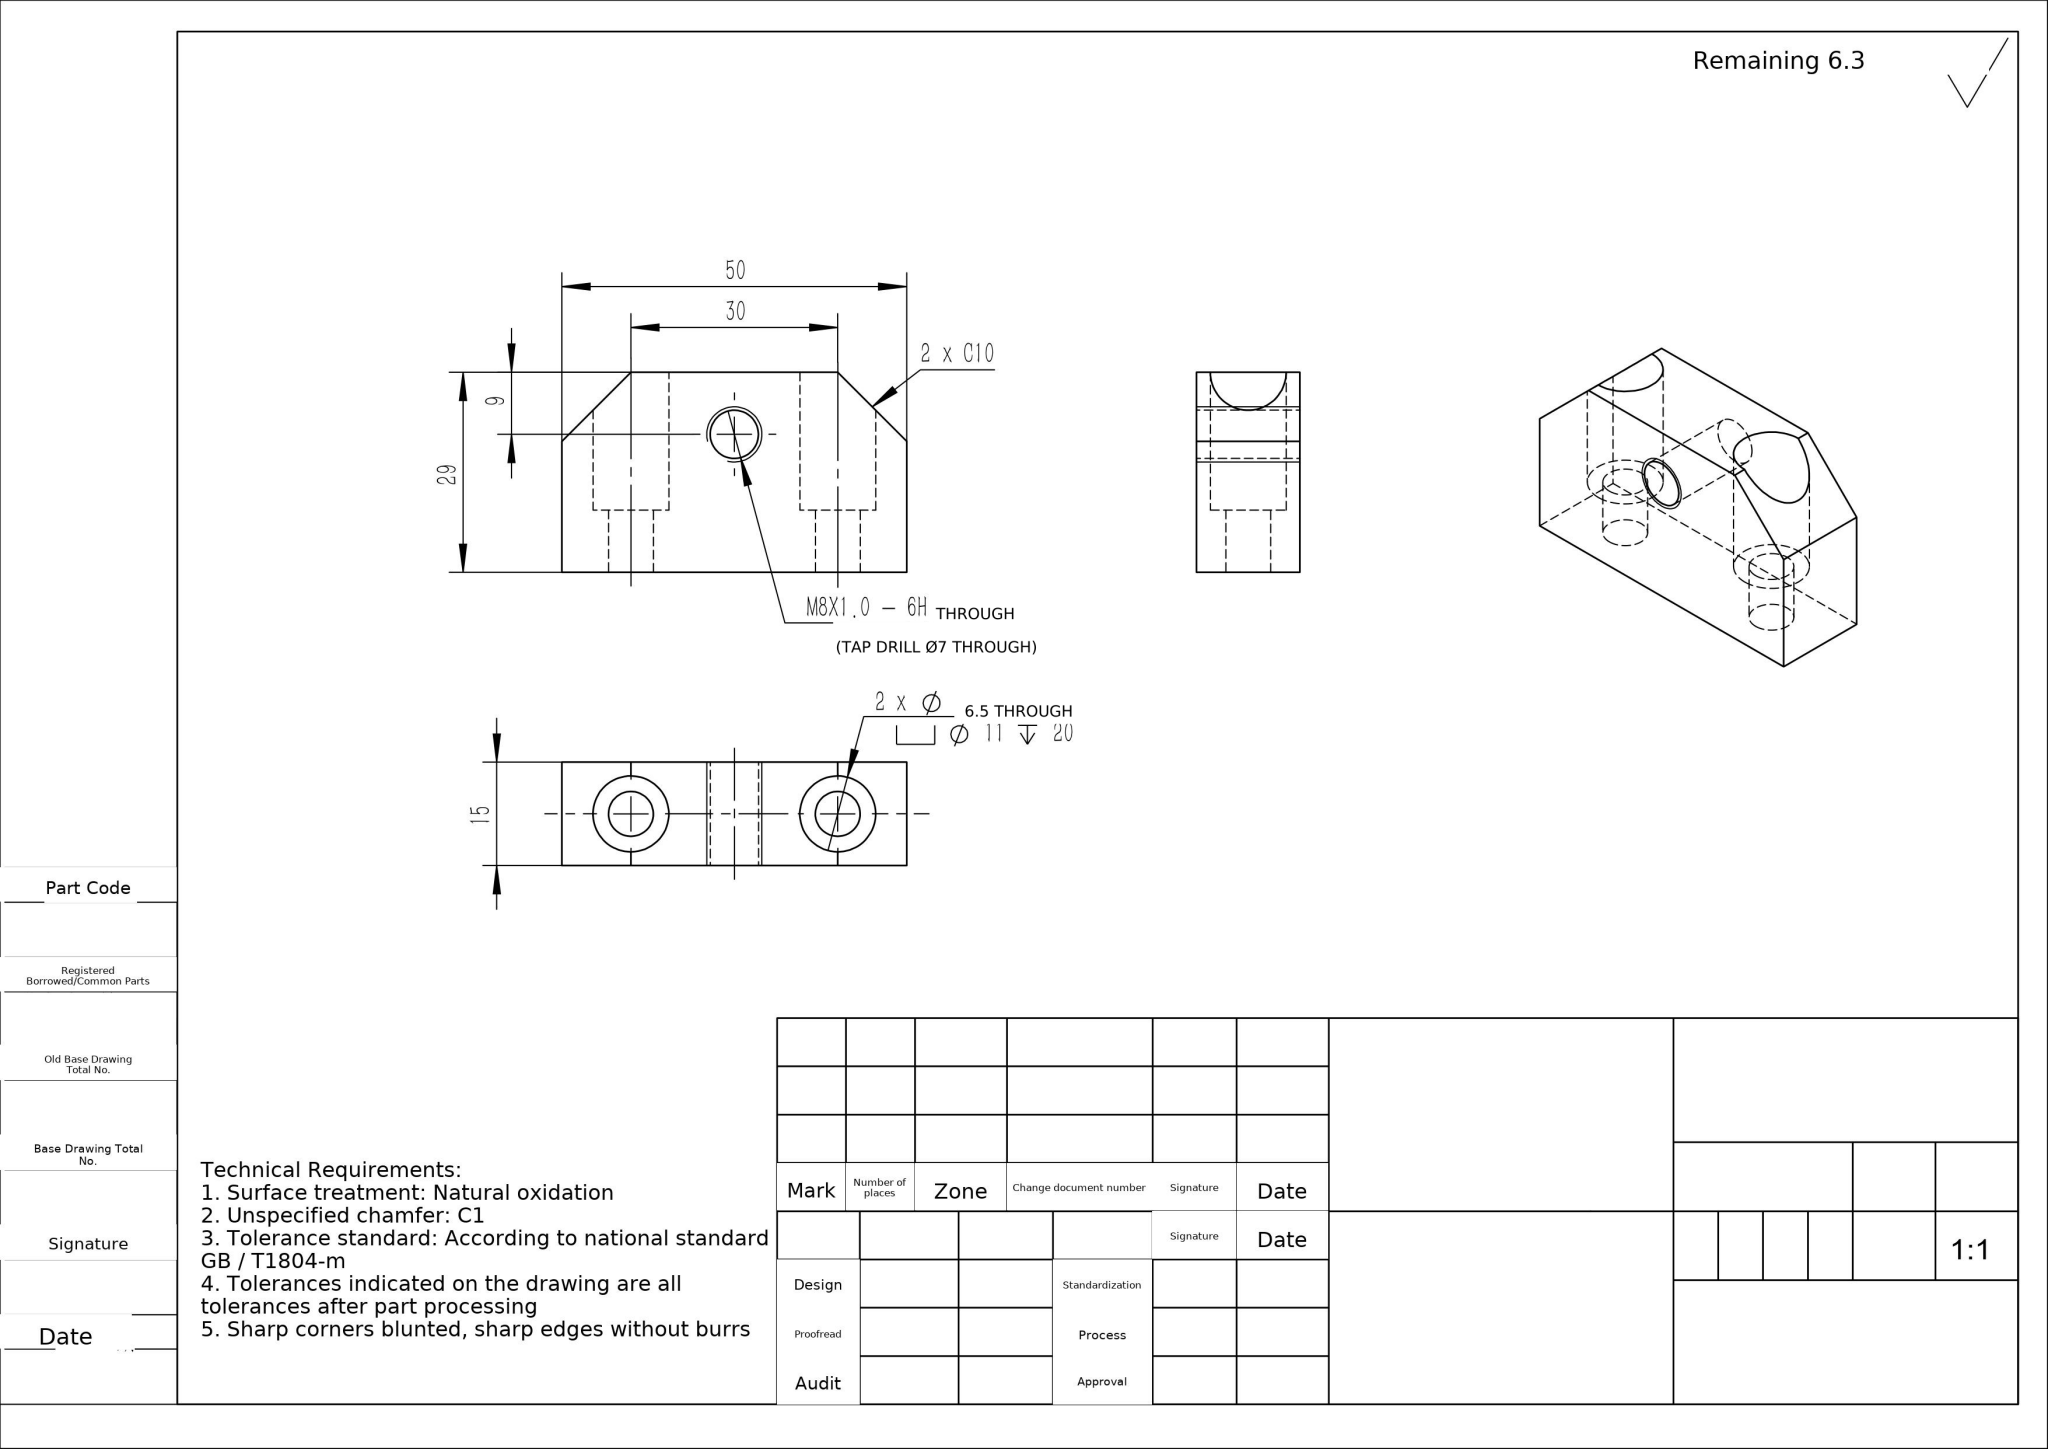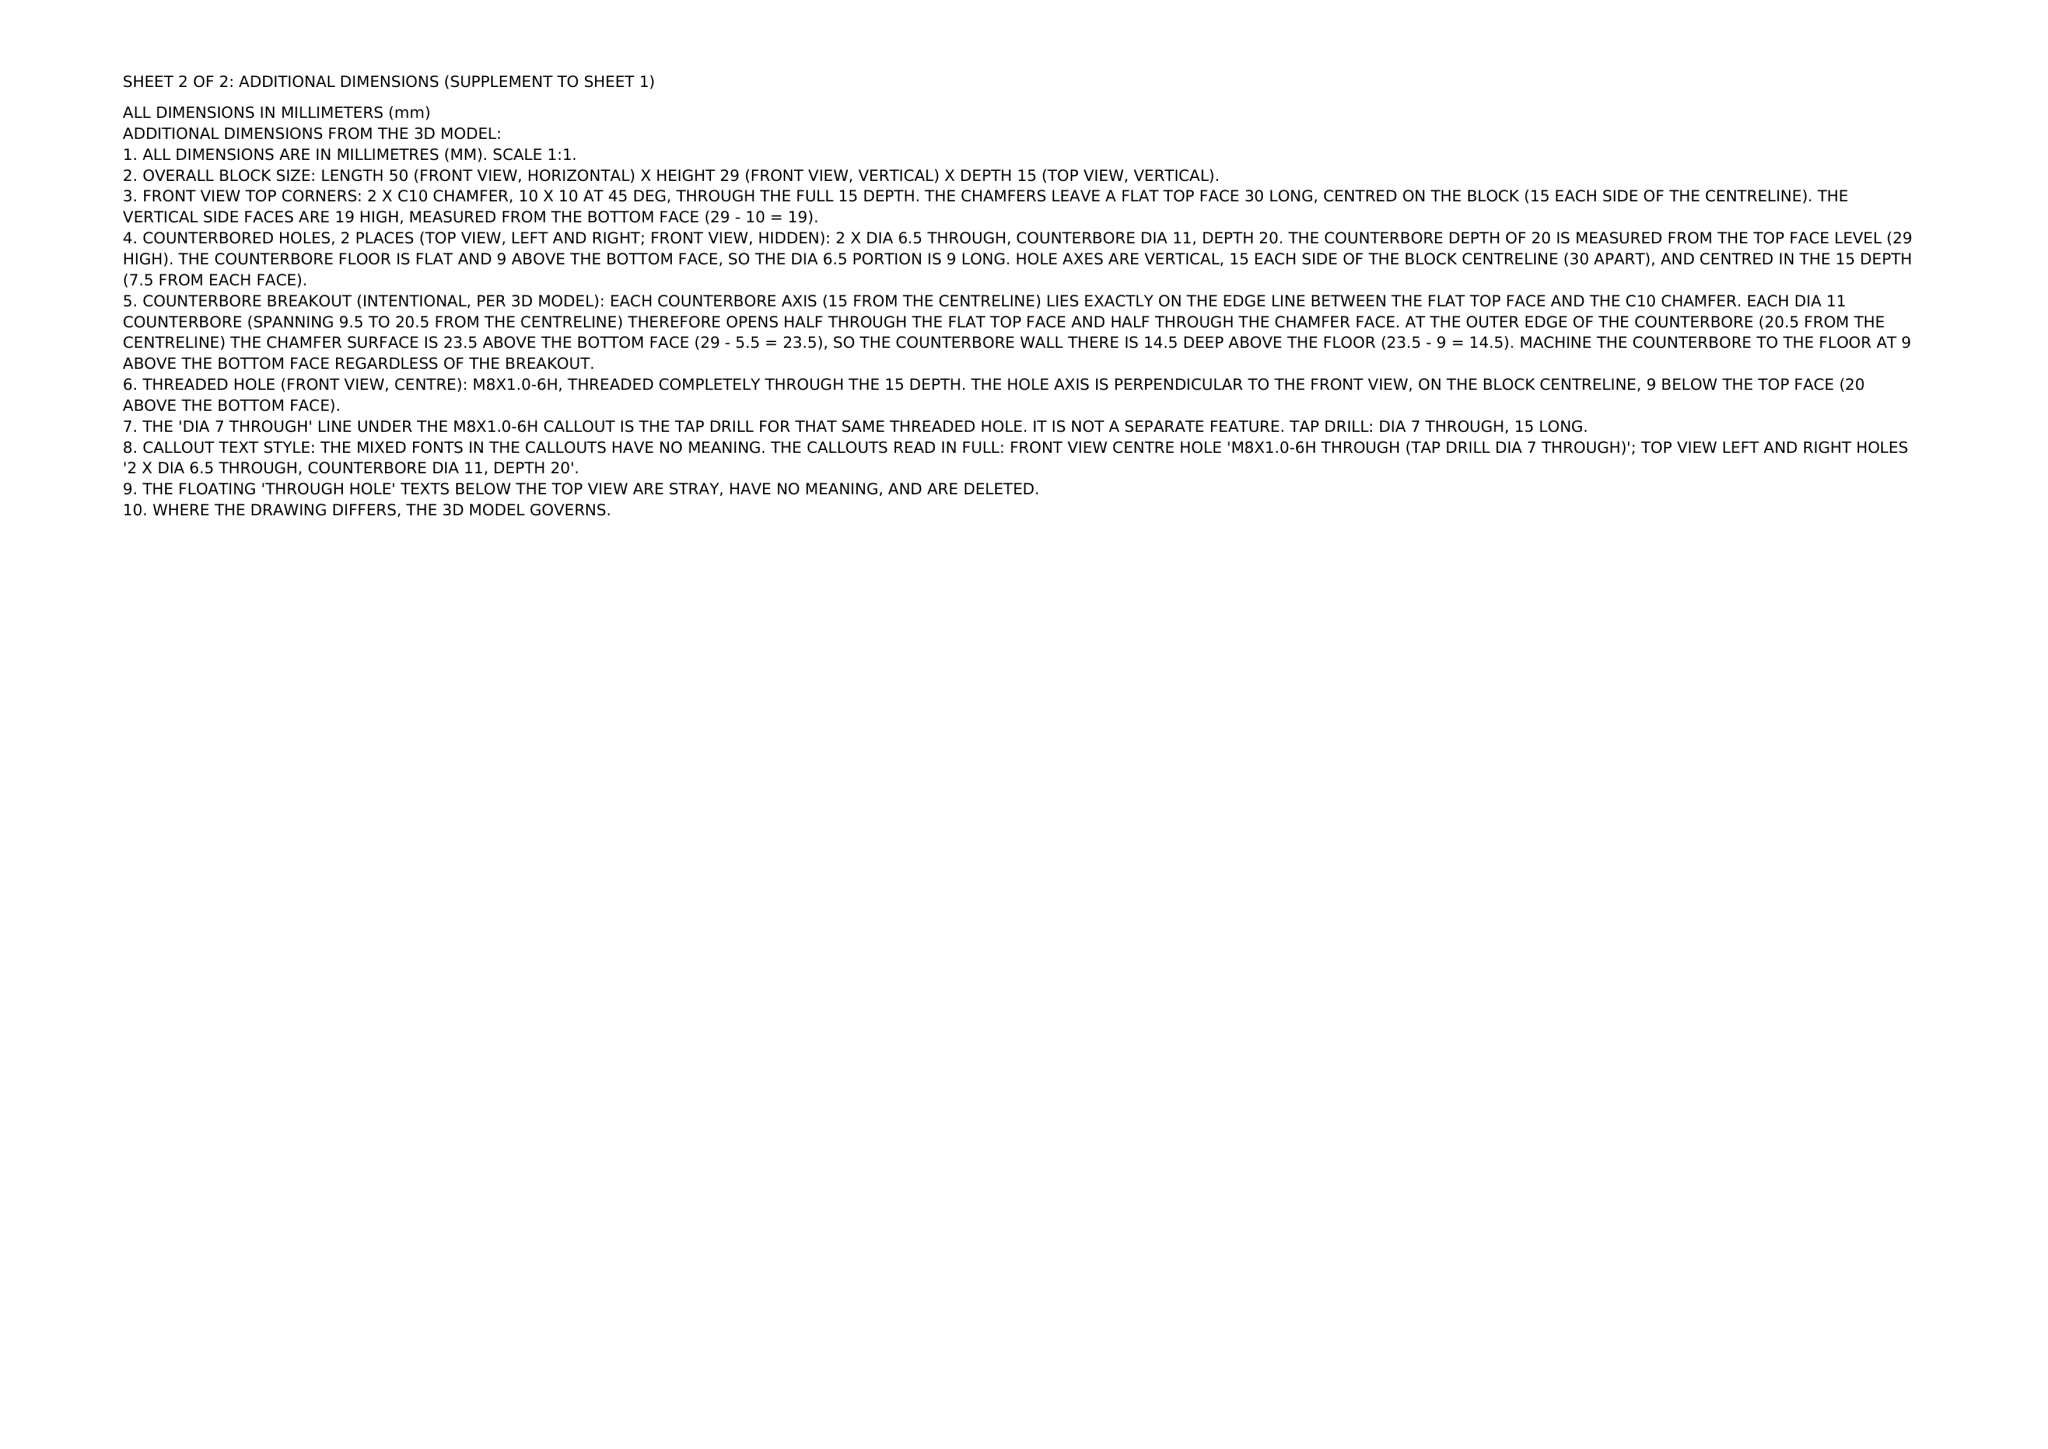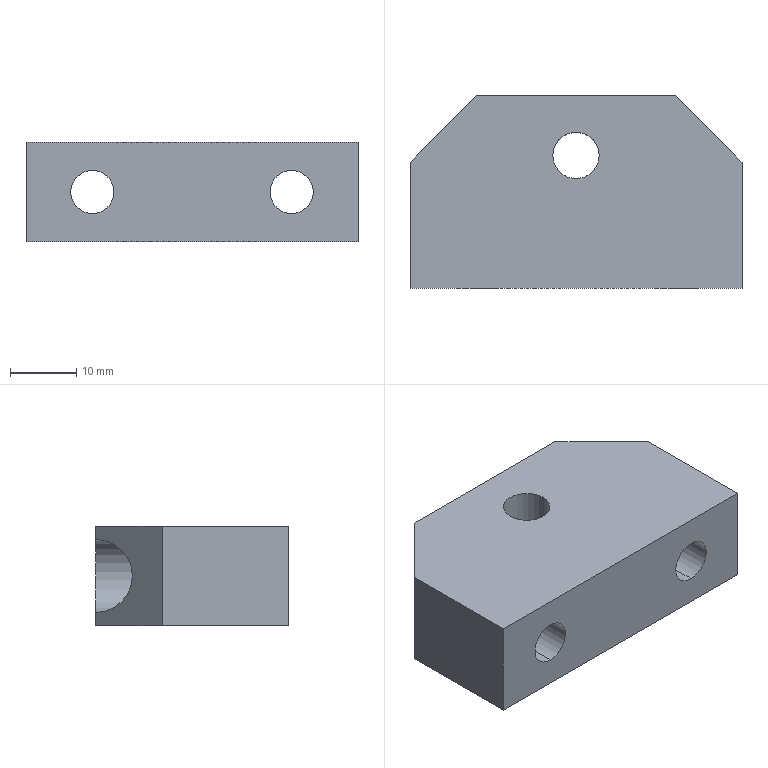Part | NX | mm | Chamfered Dual-Bore Rectangular Mounting Block | 1 solid | 20 faces | box 50 x 29 x 15 mm | volume 15496 mm3 | cylinder 10 | plane 10 | commonest cylinder face diameters 11 x4 6.5 x4 7 x2
STEP:
#1=COLOUR_RGB('',0.7922,0.8196,0.9333);
#2=FILL_AREA_STYLE_COLOUR('',#1);
#3=FILL_AREA_STYLE('',(#2));
#4=SURFACE_STYLE_FILL_AREA(#3);
#5=SURFACE_SIDE_STYLE('',(#4));
#6=SURFACE_STYLE_USAGE(.BOTH.,#5);
#7=PRESENTATION_STYLE_ASSIGNMENT((#6));
#8=CARTESIAN_POINT('',(-3.5,20.,-7.5));
#9=VERTEX_POINT('',#8);
#10=CARTESIAN_POINT('',(3.5,20.,-7.5));
#11=VERTEX_POINT('',#10);
#12=CARTESIAN_POINT('',(0.,20.,-7.5));
#13=DIRECTION('',(0.,0.,1.));
#14=DIRECTION('',(1.,0.,0.));
#15=AXIS2_PLACEMENT_3D('',#12,#13,#14);
#16=CIRCLE('',#15,3.5);
#17=EDGE_CURVE('',#9,#11,#16,.T.);
#18=ORIENTED_EDGE('',*,*,#17,.F.);
#19=CARTESIAN_POINT('',(-3.5,20.,7.5));
#20=VERTEX_POINT('',#19);
#21=CARTESIAN_POINT('',(-3.5,20.,7.5));
#22=DIRECTION('',(0.,0.,1.));
#23=VECTOR('',#22,1000.);
#24=LINE('',#21,#23);
#25=EDGE_CURVE('',#9,#20,#24,.T.);
#26=ORIENTED_EDGE('',*,*,#25,.T.);
#27=CARTESIAN_POINT('',(3.5,20.,7.5));
#28=VERTEX_POINT('',#27);
#29=CARTESIAN_POINT('',(0.,20.,7.5));
#30=DIRECTION('',(0.,0.,1.));
#31=DIRECTION('',(1.,0.,0.));
#32=AXIS2_PLACEMENT_3D('',#29,#30,#31);
#33=CIRCLE('',#32,3.5);
#34=EDGE_CURVE('',#20,#28,#33,.T.);
#35=ORIENTED_EDGE('',*,*,#34,.T.);
#36=CARTESIAN_POINT('',(3.5,20.,7.5));
#37=DIRECTION('',(0.,0.,1.));
#38=VECTOR('',#37,1000.);
#39=LINE('',#36,#38);
#40=EDGE_CURVE('',#11,#28,#39,.T.);
#41=ORIENTED_EDGE('',*,*,#40,.F.);
#42=EDGE_LOOP('',(#18,#26,#35,#41));
#43=FACE_OUTER_BOUND('',#42,.T.);
#44=CARTESIAN_POINT('',(0.,20.,7.5));
#45=DIRECTION('',(0.,0.,1.));
#46=DIRECTION('',(1.,0.,0.));
#47=AXIS2_PLACEMENT_3D('',#44,#45,#46);
#48=CYLINDRICAL_SURFACE('',#47,3.5);
#49=ADVANCED_FACE('',(#43),#48,.F.);
#50=STYLED_ITEM('',(#7),#49);
#51=PRESENTATION_LAYER_ASSIGNMENT('','',(#50));
#52=(LENGTH_UNIT()NAMED_UNIT(*)SI_UNIT(.MILLI.,.METRE.));
#53=UNCERTAINTY_MEASURE_WITH_UNIT(LENGTH_MEASURE(0.00001),#52,'','');
#54=(NAMED_UNIT(*)PLANE_ANGLE_UNIT()SI_UNIT($,.RADIAN.));
#55=(NAMED_UNIT(*)SI_UNIT($,.STERADIAN.)SOLID_ANGLE_UNIT());
#56=(GEOMETRIC_REPRESENTATION_CONTEXT(3)GLOBAL_UNCERTAINTY_ASSIGNED_CONTEXT((#53))GLOBAL_UNIT_ASSIGNED_CONTEXT((#52,#54,#55))REPRESENTATION_CONTEXT('',''));
#57=MECHANICAL_DESIGN_GEOMETRIC_PRESENTATION_REPRESENTATION('',(#50),#56);
#58=COLOUR_RGB('',0.7922,0.8196,0.9333);
#59=FILL_AREA_STYLE_COLOUR('',#58);
#60=FILL_AREA_STYLE('',(#59));
#61=SURFACE_STYLE_FILL_AREA(#60);
#62=SURFACE_SIDE_STYLE('',(#61));
#63=SURFACE_STYLE_USAGE(.BOTH.,#62);
#64=PRESENTATION_STYLE_ASSIGNMENT((#63));
#65=ORIENTED_EDGE('',*,*,#25,.F.);
#66=CARTESIAN_POINT('',(0.,20.,-7.5));
#67=DIRECTION('',(0.,0.,1.));
#68=DIRECTION('',(1.,0.,0.));
#69=AXIS2_PLACEMENT_3D('',#66,#67,#68);
#70=CIRCLE('',#69,3.5);
#71=EDGE_CURVE('',#11,#9,#70,.T.);
#72=ORIENTED_EDGE('',*,*,#71,.F.);
#73=ORIENTED_EDGE('',*,*,#40,.T.);
#74=CARTESIAN_POINT('',(0.,20.,7.5));
#75=DIRECTION('',(0.,0.,1.));
#76=DIRECTION('',(1.,0.,0.));
#77=AXIS2_PLACEMENT_3D('',#74,#75,#76);
#78=CIRCLE('',#77,3.5);
#79=EDGE_CURVE('',#28,#20,#78,.T.);
#80=ORIENTED_EDGE('',*,*,#79,.T.);
#81=EDGE_LOOP('',(#65,#72,#73,#80));
#82=FACE_OUTER_BOUND('',#81,.T.);
#83=CARTESIAN_POINT('',(0.,20.,7.5));
#84=DIRECTION('',(0.,0.,1.));
#85=DIRECTION('',(1.,0.,0.));
#86=AXIS2_PLACEMENT_3D('',#83,#84,#85);
#87=CYLINDRICAL_SURFACE('',#86,3.5);
#88=ADVANCED_FACE('',(#82),#87,.F.);
#89=STYLED_ITEM('',(#64),#88);
#90=PRESENTATION_LAYER_ASSIGNMENT('','',(#89));
#91=COLOUR_RGB('',1.,0.3725,0.6118);
#92=FILL_AREA_STYLE_COLOUR('',#91);
#93=FILL_AREA_STYLE('',(#92));
#94=SURFACE_STYLE_FILL_AREA(#93);
#95=SURFACE_SIDE_STYLE('',(#94));
#96=SURFACE_STYLE_USAGE(.BOTH.,#95);
#97=PRESENTATION_STYLE_ASSIGNMENT((#96));
#98=CARTESIAN_POINT('',(-15.,9.,-5.5));
#99=VERTEX_POINT('',#98);
#100=CARTESIAN_POINT('',(-15.,9.,5.5));
#101=VERTEX_POINT('',#100);
#102=CARTESIAN_POINT('',(-15.,9.,0.));
#103=DIRECTION('',(0.,1.,0.));
#104=DIRECTION('',(0.,0.,1.));
#105=AXIS2_PLACEMENT_3D('',#102,#103,#104);
#106=CIRCLE('',#105,5.5);
#107=EDGE_CURVE('',#99,#101,#106,.T.);
#108=ORIENTED_EDGE('',*,*,#107,.F.);
#109=CARTESIAN_POINT('',(-15.,29.,-5.5));
#110=VERTEX_POINT('',#109);
#111=CARTESIAN_POINT('',(-15.,29.,-5.5));
#112=DIRECTION('',(0.,1.,0.));
#113=VECTOR('',#112,1000.);
#114=LINE('',#111,#113);
#115=EDGE_CURVE('',#99,#110,#114,.T.);
#116=ORIENTED_EDGE('',*,*,#115,.T.);
#117=CARTESIAN_POINT('',(-15.,29.,5.5));
#118=VERTEX_POINT('',#117);
#119=CARTESIAN_POINT('',(-15.,29.,-5.5));
#120=CARTESIAN_POINT('',(-26.,18.,-5.5));
#121=CARTESIAN_POINT('',(-26.,18.,5.5));
#122=CARTESIAN_POINT('',(-15.,29.,5.5));
#123=(BOUNDED_CURVE()B_SPLINE_CURVE(3,(#119,#120,#121,#122),.UNSPECIFIED.,.F.,.T.)B_SPLINE_CURVE_WITH_KNOTS((4,4),(1.571,4.712),.UNSPECIFIED.)CURVE()GEOMETRIC_REPRESENTATION_ITEM()RATIONAL_B_SPLINE_CURVE((1.,0.3333,0.3333,1.))REPRESENTATION_ITEM(''));
#124=EDGE_CURVE('',#110,#118,#123,.T.);
#125=ORIENTED_EDGE('',*,*,#124,.T.);
#126=CARTESIAN_POINT('',(-15.,29.,5.5));
#127=DIRECTION('',(0.,1.,0.));
#128=VECTOR('',#127,1000.);
#129=LINE('',#126,#128);
#130=EDGE_CURVE('',#101,#118,#129,.T.);
#131=ORIENTED_EDGE('',*,*,#130,.F.);
#132=EDGE_LOOP('',(#108,#116,#125,#131));
#133=FACE_OUTER_BOUND('',#132,.T.);
#134=CARTESIAN_POINT('',(-15.,29.,0.));
#135=DIRECTION('',(0.,1.,0.));
#136=DIRECTION('',(0.,0.,1.));
#137=AXIS2_PLACEMENT_3D('',#134,#135,#136);
#138=CYLINDRICAL_SURFACE('',#137,5.5);
#139=ADVANCED_FACE('',(#133),#138,.F.);
#140=CARTESIAN_POINT('',(-15.,0.,-3.25));
#141=VERTEX_POINT('',#140);
#142=CARTESIAN_POINT('',(-15.,0.,3.25));
#143=VERTEX_POINT('',#142);
#144=CARTESIAN_POINT('',(-15.,0.,0.));
#145=DIRECTION('',(0.,1.,0.));
#146=DIRECTION('',(0.,0.,1.));
#147=AXIS2_PLACEMENT_3D('',#144,#145,#146);
#148=CIRCLE('',#147,3.25);
#149=EDGE_CURVE('',#141,#143,#148,.T.);
#150=ORIENTED_EDGE('',*,*,#149,.F.);
#151=CARTESIAN_POINT('',(-15.,9.,-3.25));
#152=VERTEX_POINT('',#151);
#153=CARTESIAN_POINT('',(-15.,29.,-3.25));
#154=DIRECTION('',(0.,1.,0.));
#155=VECTOR('',#154,1000.);
#156=LINE('',#153,#155);
#157=EDGE_CURVE('',#141,#152,#156,.T.);
#158=ORIENTED_EDGE('',*,*,#157,.T.);
#159=CARTESIAN_POINT('',(-15.,9.,3.25));
#160=VERTEX_POINT('',#159);
#161=CARTESIAN_POINT('',(-15.,9.,0.));
#162=DIRECTION('',(0.,1.,0.));
#163=DIRECTION('',(0.,0.,1.));
#164=AXIS2_PLACEMENT_3D('',#161,#162,#163);
#165=CIRCLE('',#164,3.25);
#166=EDGE_CURVE('',#152,#160,#165,.T.);
#167=ORIENTED_EDGE('',*,*,#166,.T.);
#168=CARTESIAN_POINT('',(-15.,29.,3.25));
#169=DIRECTION('',(0.,1.,0.));
#170=VECTOR('',#169,1000.);
#171=LINE('',#168,#170);
#172=EDGE_CURVE('',#143,#160,#171,.T.);
#173=ORIENTED_EDGE('',*,*,#172,.F.);
#174=EDGE_LOOP('',(#150,#158,#167,#173));
#175=FACE_OUTER_BOUND('',#174,.T.);
#176=CARTESIAN_POINT('',(-15.,29.,0.));
#177=DIRECTION('',(0.,1.,0.));
#178=DIRECTION('',(0.,0.,1.));
#179=AXIS2_PLACEMENT_3D('',#176,#177,#178);
#180=CYLINDRICAL_SURFACE('',#179,3.25);
#181=ADVANCED_FACE('',(#175),#180,.F.);
#182=CARTESIAN_POINT('',(15.,9.,-5.5));
#183=VERTEX_POINT('',#182);
#184=CARTESIAN_POINT('',(15.,9.,5.5));
#185=VERTEX_POINT('',#184);
#186=CARTESIAN_POINT('',(15.,9.,0.));
#187=DIRECTION('',(0.,1.,0.));
#188=DIRECTION('',(0.,0.,1.));
#189=AXIS2_PLACEMENT_3D('',#186,#187,#188);
#190=CIRCLE('',#189,5.5);
#191=EDGE_CURVE('',#183,#185,#190,.T.);
#192=ORIENTED_EDGE('',*,*,#191,.F.);
#193=CARTESIAN_POINT('',(15.,29.,-5.5));
#194=VERTEX_POINT('',#193);
#195=CARTESIAN_POINT('',(15.,29.,-5.5));
#196=DIRECTION('',(0.,1.,0.));
#197=VECTOR('',#196,1000.);
#198=LINE('',#195,#197);
#199=EDGE_CURVE('',#183,#194,#198,.T.);
#200=ORIENTED_EDGE('',*,*,#199,.T.);
#201=CARTESIAN_POINT('',(15.,29.,5.5));
#202=VERTEX_POINT('',#201);
#203=CARTESIAN_POINT('',(15.,29.,0.));
#204=DIRECTION('',(0.,1.,0.));
#205=DIRECTION('',(0.,0.,1.));
#206=AXIS2_PLACEMENT_3D('',#203,#204,#205);
#207=CIRCLE('',#206,5.5);
#208=EDGE_CURVE('',#194,#202,#207,.T.);
#209=ORIENTED_EDGE('',*,*,#208,.T.);
#210=CARTESIAN_POINT('',(15.,29.,5.5));
#211=DIRECTION('',(0.,1.,0.));
#212=VECTOR('',#211,1000.);
#213=LINE('',#210,#212);
#214=EDGE_CURVE('',#185,#202,#213,.T.);
#215=ORIENTED_EDGE('',*,*,#214,.F.);
#216=EDGE_LOOP('',(#192,#200,#209,#215));
#217=FACE_OUTER_BOUND('',#216,.T.);
#218=CARTESIAN_POINT('',(15.,29.,0.));
#219=DIRECTION('',(0.,1.,0.));
#220=DIRECTION('',(0.,0.,1.));
#221=AXIS2_PLACEMENT_3D('',#218,#219,#220);
#222=CYLINDRICAL_SURFACE('',#221,5.5);
#223=ADVANCED_FACE('',(#217),#222,.F.);
#224=CARTESIAN_POINT('',(15.,0.,-3.25));
#225=VERTEX_POINT('',#224);
#226=CARTESIAN_POINT('',(15.,0.,3.25));
#227=VERTEX_POINT('',#226);
#228=CARTESIAN_POINT('',(15.,0.,0.));
#229=DIRECTION('',(0.,1.,0.));
#230=DIRECTION('',(0.,0.,1.));
#231=AXIS2_PLACEMENT_3D('',#228,#229,#230);
#232=CIRCLE('',#231,3.25);
#233=EDGE_CURVE('',#225,#227,#232,.T.);
#234=ORIENTED_EDGE('',*,*,#233,.F.);
#235=CARTESIAN_POINT('',(15.,9.,-3.25));
#236=VERTEX_POINT('',#235);
#237=CARTESIAN_POINT('',(15.,29.,-3.25));
#238=DIRECTION('',(0.,1.,0.));
#239=VECTOR('',#238,1000.);
#240=LINE('',#237,#239);
#241=EDGE_CURVE('',#225,#236,#240,.T.);
#242=ORIENTED_EDGE('',*,*,#241,.T.);
#243=CARTESIAN_POINT('',(15.,9.,3.25));
#244=VERTEX_POINT('',#243);
#245=CARTESIAN_POINT('',(15.,9.,0.));
#246=DIRECTION('',(0.,1.,0.));
#247=DIRECTION('',(0.,0.,1.));
#248=AXIS2_PLACEMENT_3D('',#245,#246,#247);
#249=CIRCLE('',#248,3.25);
#250=EDGE_CURVE('',#236,#244,#249,.T.);
#251=ORIENTED_EDGE('',*,*,#250,.T.);
#252=CARTESIAN_POINT('',(15.,29.,3.25));
#253=DIRECTION('',(0.,1.,0.));
#254=VECTOR('',#253,1000.);
#255=LINE('',#252,#254);
#256=EDGE_CURVE('',#227,#244,#255,.T.);
#257=ORIENTED_EDGE('',*,*,#256,.F.);
#258=EDGE_LOOP('',(#234,#242,#251,#257));
#259=FACE_OUTER_BOUND('',#258,.T.);
#260=CARTESIAN_POINT('',(15.,29.,0.));
#261=DIRECTION('',(0.,1.,0.));
#262=DIRECTION('',(0.,0.,1.));
#263=AXIS2_PLACEMENT_3D('',#260,#261,#262);
#264=CYLINDRICAL_SURFACE('',#263,3.25);
#265=ADVANCED_FACE('',(#259),#264,.F.);
#266=CARTESIAN_POINT('',(25.,19.,-7.5));
#267=VERTEX_POINT('',#266);
#268=CARTESIAN_POINT('',(25.,0.,-7.5));
#269=VERTEX_POINT('',#268);
#270=CARTESIAN_POINT('',(25.,29.,-7.5));
#271=DIRECTION('',(0.,-1.,0.));
#272=VECTOR('',#271,1000.);
#273=LINE('',#270,#272);
#274=EDGE_CURVE('',#267,#269,#273,.T.);
#275=ORIENTED_EDGE('',*,*,#274,.F.);
#276=CARTESIAN_POINT('',(25.,19.,7.5));
#277=VERTEX_POINT('',#276);
#278=CARTESIAN_POINT('',(25.,19.,7.5));
#279=DIRECTION('',(0.,0.,1.));
#280=VECTOR('',#279,1000.);
#281=LINE('',#278,#280);
#282=EDGE_CURVE('',#267,#277,#281,.T.);
#283=ORIENTED_EDGE('',*,*,#282,.T.);
#284=CARTESIAN_POINT('',(25.,0.,7.5));
#285=VERTEX_POINT('',#284);
#286=CARTESIAN_POINT('',(25.,29.,7.5));
#287=DIRECTION('',(0.,-1.,0.));
#288=VECTOR('',#287,1000.);
#289=LINE('',#286,#288);
#290=EDGE_CURVE('',#277,#285,#289,.T.);
#291=ORIENTED_EDGE('',*,*,#290,.T.);
#292=CARTESIAN_POINT('',(25.,0.,7.5));
#293=DIRECTION('',(0.,0.,-1.));
#294=VECTOR('',#293,1000.);
#295=LINE('',#292,#294);
#296=EDGE_CURVE('',#285,#269,#295,.T.);
#297=ORIENTED_EDGE('',*,*,#296,.T.);
#298=EDGE_LOOP('',(#275,#283,#291,#297));
#299=FACE_OUTER_BOUND('',#298,.T.);
#300=CARTESIAN_POINT('',(25.,29.,7.5));
#301=DIRECTION('',(-1.,0.,0.));
#302=DIRECTION('',(0.,0.,1.));
#303=AXIS2_PLACEMENT_3D('',#300,#301,#302);
#304=PLANE('',#303);
#305=ADVANCED_FACE('',(#299),#304,.F.);
#306=ORIENTED_EDGE('',*,*,#71,.T.);
#307=ORIENTED_EDGE('',*,*,#17,.T.);
#308=EDGE_LOOP('',(#306,#307));
#309=FACE_BOUND('',#308,.T.);
#310=CARTESIAN_POINT('',(-25.,19.,-7.5));
#311=VERTEX_POINT('',#310);
#312=CARTESIAN_POINT('',(-25.,0.,-7.5));
#313=VERTEX_POINT('',#312);
#314=CARTESIAN_POINT('',(-25.,29.,-7.5));
#315=DIRECTION('',(0.,-1.,0.));
#316=VECTOR('',#315,1000.);
#317=LINE('',#314,#316);
#318=EDGE_CURVE('',#311,#313,#317,.T.);
#319=ORIENTED_EDGE('',*,*,#318,.F.);
#320=CARTESIAN_POINT('',(-15.,29.,-7.5));
#321=VERTEX_POINT('',#320);
#322=CARTESIAN_POINT('',(-15.,29.,-7.5));
#323=DIRECTION('',(0.7071,0.7071,0.));
#324=VECTOR('',#323,1000.);
#325=LINE('',#322,#324);
#326=EDGE_CURVE('',#311,#321,#325,.T.);
#327=ORIENTED_EDGE('',*,*,#326,.T.);
#328=CARTESIAN_POINT('',(15.,29.,-7.5));
#329=VERTEX_POINT('',#328);
#330=CARTESIAN_POINT('',(-25.,29.,-7.5));
#331=DIRECTION('',(-1.,0.,0.));
#332=VECTOR('',#331,1000.);
#333=LINE('',#330,#332);
#334=EDGE_CURVE('',#329,#321,#333,.T.);
#335=ORIENTED_EDGE('',*,*,#334,.F.);
#336=CARTESIAN_POINT('',(15.,29.,-7.5));
#337=DIRECTION('',(0.7071,-0.7071,0.));
#338=VECTOR('',#337,1000.);
#339=LINE('',#336,#338);
#340=EDGE_CURVE('',#329,#267,#339,.T.);
#341=ORIENTED_EDGE('',*,*,#340,.T.);
#342=ORIENTED_EDGE('',*,*,#274,.T.);
#343=CARTESIAN_POINT('',(-25.,0.,-7.5));
#344=DIRECTION('',(-1.,0.,0.));
#345=VECTOR('',#344,1000.);
#346=LINE('',#343,#345);
#347=EDGE_CURVE('',#269,#313,#346,.T.);
#348=ORIENTED_EDGE('',*,*,#347,.T.);
#349=EDGE_LOOP('',(#319,#327,#335,#341,#342,#348));
#350=FACE_OUTER_BOUND('',#349,.T.);
#351=CARTESIAN_POINT('',(-25.,29.,-7.5));
#352=DIRECTION('',(0.,0.,1.));
#353=DIRECTION('',(1.,0.,0.));
#354=AXIS2_PLACEMENT_3D('',#351,#352,#353);
#355=PLANE('',#354);
#356=ADVANCED_FACE('',(#309,#350),#355,.F.);
#357=CARTESIAN_POINT('',(-25.,19.,7.5));
#358=VERTEX_POINT('',#357);
#359=CARTESIAN_POINT('',(-25.,0.,7.5));
#360=VERTEX_POINT('',#359);
#361=CARTESIAN_POINT('',(-25.,29.,7.5));
#362=DIRECTION('',(0.,-1.,0.));
#363=VECTOR('',#362,1000.);
#364=LINE('',#361,#363);
#365=EDGE_CURVE('',#358,#360,#364,.T.);
#366=ORIENTED_EDGE('',*,*,#365,.F.);
#367=CARTESIAN_POINT('',(-25.,19.,7.5));
#368=DIRECTION('',(0.,0.,-1.));
#369=VECTOR('',#368,1000.);
#370=LINE('',#367,#369);
#371=EDGE_CURVE('',#358,#311,#370,.T.);
#372=ORIENTED_EDGE('',*,*,#371,.T.);
#373=ORIENTED_EDGE('',*,*,#318,.T.);
#374=CARTESIAN_POINT('',(-25.,0.,7.5));
#375=DIRECTION('',(0.,0.,1.));
#376=VECTOR('',#375,1000.);
#377=LINE('',#374,#376);
#378=EDGE_CURVE('',#313,#360,#377,.T.);
#379=ORIENTED_EDGE('',*,*,#378,.T.);
#380=EDGE_LOOP('',(#366,#372,#373,#379));
#381=FACE_OUTER_BOUND('',#380,.T.);
#382=CARTESIAN_POINT('',(-25.,29.,7.5));
#383=DIRECTION('',(1.,0.,0.));
#384=DIRECTION('',(0.,0.,-1.));
#385=AXIS2_PLACEMENT_3D('',#382,#383,#384);
#386=PLANE('',#385);
#387=ADVANCED_FACE('',(#381),#386,.F.);
#388=ORIENTED_EDGE('',*,*,#79,.F.);
#389=ORIENTED_EDGE('',*,*,#34,.F.);
#390=EDGE_LOOP('',(#388,#389));
#391=FACE_BOUND('',#390,.T.);
#392=CARTESIAN_POINT('',(-15.,29.,7.5));
#393=VERTEX_POINT('',#392);
#394=CARTESIAN_POINT('',(15.,29.,7.5));
#395=VERTEX_POINT('',#394);
#396=CARTESIAN_POINT('',(-25.,29.,7.5));
#397=DIRECTION('',(1.,0.,0.));
#398=VECTOR('',#397,1000.);
#399=LINE('',#396,#398);
#400=EDGE_CURVE('',#393,#395,#399,.T.);
#401=ORIENTED_EDGE('',*,*,#400,.F.);
#402=CARTESIAN_POINT('',(-15.,29.,7.5));
#403=DIRECTION('',(-0.7071,-0.7071,0.));
#404=VECTOR('',#403,1000.);
#405=LINE('',#402,#404);
#406=EDGE_CURVE('',#393,#358,#405,.T.);
#407=ORIENTED_EDGE('',*,*,#406,.T.);
#408=ORIENTED_EDGE('',*,*,#365,.T.);
#409=CARTESIAN_POINT('',(-25.,0.,7.5));
#410=DIRECTION('',(1.,0.,0.));
#411=VECTOR('',#410,1000.);
#412=LINE('',#409,#411);
#413=EDGE_CURVE('',#360,#285,#412,.T.);
#414=ORIENTED_EDGE('',*,*,#413,.T.);
#415=ORIENTED_EDGE('',*,*,#290,.F.);
#416=CARTESIAN_POINT('',(15.,29.,7.5));
#417=DIRECTION('',(-0.7071,0.7071,0.));
#418=VECTOR('',#417,1000.);
#419=LINE('',#416,#418);
#420=EDGE_CURVE('',#277,#395,#419,.T.);
#421=ORIENTED_EDGE('',*,*,#420,.T.);
#422=EDGE_LOOP('',(#401,#407,#408,#414,#415,#421));
#423=FACE_OUTER_BOUND('',#422,.T.);
#424=CARTESIAN_POINT('',(-25.,29.,7.5));
#425=DIRECTION('',(0.,0.,-1.));
#426=DIRECTION('',(-1.,0.,0.));
#427=AXIS2_PLACEMENT_3D('',#424,#425,#426);
#428=PLANE('',#427);
#429=ADVANCED_FACE('',(#391,#423),#428,.F.);
#430=ORIENTED_EDGE('',*,*,#334,.T.);
#431=CARTESIAN_POINT('',(-15.,29.,0.));
#432=DIRECTION('',(0.,0.,1.));
#433=VECTOR('',#432,1000.);
#434=LINE('',#431,#433);
#435=EDGE_CURVE('',#321,#110,#434,.T.);
#436=ORIENTED_EDGE('',*,*,#435,.T.);
#437=CARTESIAN_POINT('',(-15.,29.,0.));
#438=DIRECTION('',(0.,1.,0.));
#439=DIRECTION('',(0.,0.,1.));
#440=AXIS2_PLACEMENT_3D('',#437,#438,#439);
#441=CIRCLE('',#440,5.5);
#442=EDGE_CURVE('',#118,#110,#441,.T.);
#443=ORIENTED_EDGE('',*,*,#442,.F.);
#444=CARTESIAN_POINT('',(-15.,29.,0.));
#445=DIRECTION('',(0.,0.,1.));
#446=VECTOR('',#445,1000.);
#447=LINE('',#444,#446);
#448=EDGE_CURVE('',#118,#393,#447,.T.);
#449=ORIENTED_EDGE('',*,*,#448,.T.);
#450=ORIENTED_EDGE('',*,*,#400,.T.);
#451=CARTESIAN_POINT('',(15.,29.,0.));
#452=DIRECTION('',(0.,0.,-1.));
#453=VECTOR('',#452,1000.);
#454=LINE('',#451,#453);
#455=EDGE_CURVE('',#395,#202,#454,.T.);
#456=ORIENTED_EDGE('',*,*,#455,.T.);
#457=ORIENTED_EDGE('',*,*,#208,.F.);
#458=CARTESIAN_POINT('',(15.,29.,0.));
#459=DIRECTION('',(0.,0.,-1.));
#460=VECTOR('',#459,1000.);
#461=LINE('',#458,#460);
#462=EDGE_CURVE('',#194,#329,#461,.T.);
#463=ORIENTED_EDGE('',*,*,#462,.T.);
#464=EDGE_LOOP('',(#430,#436,#443,#449,#450,#456,#457,#463));
#465=FACE_OUTER_BOUND('',#464,.T.);
#466=CARTESIAN_POINT('',(0.,29.,0.));
#467=DIRECTION('',(0.,-1.,0.));
#468=DIRECTION('',(0.,0.,-1.));
#469=AXIS2_PLACEMENT_3D('',#466,#467,#468);
#470=PLANE('',#469);
#471=ADVANCED_FACE('',(#465),#470,.F.);
#472=CARTESIAN_POINT('',(-15.,0.,0.));
#473=DIRECTION('',(0.,1.,0.));
#474=DIRECTION('',(0.,0.,1.));
#475=AXIS2_PLACEMENT_3D('',#472,#473,#474);
#476=CIRCLE('',#475,3.25);
#477=EDGE_CURVE('',#143,#141,#476,.T.);
#478=ORIENTED_EDGE('',*,*,#477,.T.);
#479=ORIENTED_EDGE('',*,*,#149,.T.);
#480=EDGE_LOOP('',(#478,#479));
#481=FACE_BOUND('',#480,.T.);
#482=CARTESIAN_POINT('',(15.,0.,0.));
#483=DIRECTION('',(0.,1.,0.));
#484=DIRECTION('',(0.,0.,1.));
#485=AXIS2_PLACEMENT_3D('',#482,#483,#484);
#486=CIRCLE('',#485,3.25);
#487=EDGE_CURVE('',#227,#225,#486,.T.);
#488=ORIENTED_EDGE('',*,*,#487,.T.);
#489=ORIENTED_EDGE('',*,*,#233,.T.);
#490=EDGE_LOOP('',(#488,#489));
#491=FACE_BOUND('',#490,.T.);
#492=ORIENTED_EDGE('',*,*,#296,.F.);
#493=ORIENTED_EDGE('',*,*,#413,.F.);
#494=ORIENTED_EDGE('',*,*,#378,.F.);
#495=ORIENTED_EDGE('',*,*,#347,.F.);
#496=EDGE_LOOP('',(#492,#493,#494,#495));
#497=FACE_OUTER_BOUND('',#496,.T.);
#498=CARTESIAN_POINT('',(0.,0.,0.));
#499=DIRECTION('',(0.,-1.,0.));
#500=DIRECTION('',(0.,0.,-1.));
#501=AXIS2_PLACEMENT_3D('',#498,#499,#500);
#502=PLANE('',#501);
#503=ADVANCED_FACE('',(#481,#491,#497),#502,.T.);
#504=ORIENTED_EDGE('',*,*,#241,.F.);
#505=ORIENTED_EDGE('',*,*,#487,.F.);
#506=ORIENTED_EDGE('',*,*,#256,.T.);
#507=CARTESIAN_POINT('',(15.,9.,0.));
#508=DIRECTION('',(0.,1.,0.));
#509=DIRECTION('',(0.,0.,1.));
#510=AXIS2_PLACEMENT_3D('',#507,#508,#509);
#511=CIRCLE('',#510,3.25);
#512=EDGE_CURVE('',#244,#236,#511,.T.);
#513=ORIENTED_EDGE('',*,*,#512,.T.);
#514=EDGE_LOOP('',(#504,#505,#506,#513));
#515=FACE_OUTER_BOUND('',#514,.T.);
#516=CARTESIAN_POINT('',(15.,29.,0.));
#517=DIRECTION('',(0.,1.,0.));
#518=DIRECTION('',(0.,0.,1.));
#519=AXIS2_PLACEMENT_3D('',#516,#517,#518);
#520=CYLINDRICAL_SURFACE('',#519,3.25);
#521=ADVANCED_FACE('',(#515),#520,.F.);
#522=ORIENTED_EDGE('',*,*,#512,.F.);
#523=ORIENTED_EDGE('',*,*,#250,.F.);
#524=EDGE_LOOP('',(#522,#523));
#525=FACE_BOUND('',#524,.T.);
#526=CARTESIAN_POINT('',(15.,9.,0.));
#527=DIRECTION('',(0.,1.,0.));
#528=DIRECTION('',(0.,0.,1.));
#529=AXIS2_PLACEMENT_3D('',#526,#527,#528);
#530=CIRCLE('',#529,5.5);
#531=EDGE_CURVE('',#185,#183,#530,.T.);
#532=ORIENTED_EDGE('',*,*,#531,.T.);
#533=ORIENTED_EDGE('',*,*,#191,.T.);
#534=EDGE_LOOP('',(#532,#533));
#535=FACE_OUTER_BOUND('',#534,.T.);
#536=CARTESIAN_POINT('',(18.25,9.,0.));
#537=DIRECTION('',(0.,-1.,0.));
#538=DIRECTION('',(0.,0.,-1.));
#539=AXIS2_PLACEMENT_3D('',#536,#537,#538);
#540=PLANE('',#539);
#541=ADVANCED_FACE('',(#525,#535),#540,.F.);
#542=ORIENTED_EDGE('',*,*,#199,.F.);
#543=ORIENTED_EDGE('',*,*,#531,.F.);
#544=ORIENTED_EDGE('',*,*,#214,.T.);
#545=CARTESIAN_POINT('',(15.,29.,5.5));
#546=CARTESIAN_POINT('',(26.,18.,5.5));
#547=CARTESIAN_POINT('',(26.,18.,-5.5));
#548=CARTESIAN_POINT('',(15.,29.,-5.5));
#549=(BOUNDED_CURVE()B_SPLINE_CURVE(3,(#545,#546,#547,#548),.UNSPECIFIED.,.F.,.T.)B_SPLINE_CURVE_WITH_KNOTS((4,4),(1.571,4.712),.UNSPECIFIED.)CURVE()GEOMETRIC_REPRESENTATION_ITEM()RATIONAL_B_SPLINE_CURVE((1.,0.3333,0.3333,1.))REPRESENTATION_ITEM(''));
#550=EDGE_CURVE('',#202,#194,#549,.T.);
#551=ORIENTED_EDGE('',*,*,#550,.T.);
#552=EDGE_LOOP('',(#542,#543,#544,#551));
#553=FACE_OUTER_BOUND('',#552,.T.);
#554=CARTESIAN_POINT('',(15.,29.,0.));
#555=DIRECTION('',(0.,1.,0.));
#556=DIRECTION('',(0.,0.,1.));
#557=AXIS2_PLACEMENT_3D('',#554,#555,#556);
#558=CYLINDRICAL_SURFACE('',#557,5.5);
#559=ADVANCED_FACE('',(#553),#558,.F.);
#560=ORIENTED_EDGE('',*,*,#157,.F.);
#561=ORIENTED_EDGE('',*,*,#477,.F.);
#562=ORIENTED_EDGE('',*,*,#172,.T.);
#563=CARTESIAN_POINT('',(-15.,9.,0.));
#564=DIRECTION('',(0.,1.,0.));
#565=DIRECTION('',(0.,0.,1.));
#566=AXIS2_PLACEMENT_3D('',#563,#564,#565);
#567=CIRCLE('',#566,3.25);
#568=EDGE_CURVE('',#160,#152,#567,.T.);
#569=ORIENTED_EDGE('',*,*,#568,.T.);
#570=EDGE_LOOP('',(#560,#561,#562,#569));
#571=FACE_OUTER_BOUND('',#570,.T.);
#572=CARTESIAN_POINT('',(-15.,29.,0.));
#573=DIRECTION('',(0.,1.,0.));
#574=DIRECTION('',(0.,0.,1.));
#575=AXIS2_PLACEMENT_3D('',#572,#573,#574);
#576=CYLINDRICAL_SURFACE('',#575,3.25);
#577=ADVANCED_FACE('',(#571),#576,.F.);
#578=ORIENTED_EDGE('',*,*,#568,.F.);
#579=ORIENTED_EDGE('',*,*,#166,.F.);
#580=EDGE_LOOP('',(#578,#579));
#581=FACE_BOUND('',#580,.T.);
#582=CARTESIAN_POINT('',(-15.,9.,0.));
#583=DIRECTION('',(0.,1.,0.));
#584=DIRECTION('',(0.,0.,1.));
#585=AXIS2_PLACEMENT_3D('',#582,#583,#584);
#586=CIRCLE('',#585,5.5);
#587=EDGE_CURVE('',#101,#99,#586,.T.);
#588=ORIENTED_EDGE('',*,*,#587,.T.);
#589=ORIENTED_EDGE('',*,*,#107,.T.);
#590=EDGE_LOOP('',(#588,#589));
#591=FACE_OUTER_BOUND('',#590,.T.);
#592=CARTESIAN_POINT('',(-11.75,9.,0.));
#593=DIRECTION('',(0.,-1.,0.));
#594=DIRECTION('',(0.,0.,-1.));
#595=AXIS2_PLACEMENT_3D('',#592,#593,#594);
#596=PLANE('',#595);
#597=ADVANCED_FACE('',(#581,#591),#596,.F.);
#598=ORIENTED_EDGE('',*,*,#115,.F.);
#599=ORIENTED_EDGE('',*,*,#587,.F.);
#600=ORIENTED_EDGE('',*,*,#130,.T.);
#601=ORIENTED_EDGE('',*,*,#442,.T.);
#602=EDGE_LOOP('',(#598,#599,#600,#601));
#603=FACE_OUTER_BOUND('',#602,.T.);
#604=CARTESIAN_POINT('',(-15.,29.,0.));
#605=DIRECTION('',(0.,1.,0.));
#606=DIRECTION('',(0.,0.,1.));
#607=AXIS2_PLACEMENT_3D('',#604,#605,#606);
#608=CYLINDRICAL_SURFACE('',#607,5.5);
#609=ADVANCED_FACE('',(#603),#608,.F.);
#610=ORIENTED_EDGE('',*,*,#326,.F.);
#611=ORIENTED_EDGE('',*,*,#371,.F.);
#612=ORIENTED_EDGE('',*,*,#406,.F.);
#613=ORIENTED_EDGE('',*,*,#448,.F.);
#614=ORIENTED_EDGE('',*,*,#124,.F.);
#615=ORIENTED_EDGE('',*,*,#435,.F.);
#616=EDGE_LOOP('',(#610,#611,#612,#613,#614,#615));
#617=FACE_OUTER_BOUND('',#616,.T.);
#618=CARTESIAN_POINT('',(-15.,29.,0.));
#619=DIRECTION('',(0.7071,-0.7071,0.));
#620=DIRECTION('',(0.,0.,1.));
#621=AXIS2_PLACEMENT_3D('',#618,#619,#620);
#622=PLANE('',#621);
#623=ADVANCED_FACE('',(#617),#622,.F.);
#624=ORIENTED_EDGE('',*,*,#420,.F.);
#625=ORIENTED_EDGE('',*,*,#282,.F.);
#626=ORIENTED_EDGE('',*,*,#340,.F.);
#627=ORIENTED_EDGE('',*,*,#462,.F.);
#628=ORIENTED_EDGE('',*,*,#550,.F.);
#629=ORIENTED_EDGE('',*,*,#455,.F.);
#630=EDGE_LOOP('',(#624,#625,#626,#627,#628,#629));
#631=FACE_OUTER_BOUND('',#630,.T.);
#632=CARTESIAN_POINT('',(15.,29.,0.));
#633=DIRECTION('',(-0.7071,-0.7071,0.));
#634=DIRECTION('',(0.,0.,-1.));
#635=AXIS2_PLACEMENT_3D('',#632,#633,#634);
#636=PLANE('',#635);
#637=ADVANCED_FACE('',(#631),#636,.F.);
#638=CLOSED_SHELL('',(#49,#139,#181,#223,#265,#305,#356,#387,#429,#471,#503,#521,#541,#559,#577,#597,#609,#88,#623,#637));
#639=MANIFOLD_SOLID_BREP('',#638);
#640=CARTESIAN_POINT('',(0.,0.,0.));
#641=DIRECTION('',(0.,0.,1.));
#642=DIRECTION('',(1.,0.,0.));
#643=AXIS2_PLACEMENT_3D('',#640,#641,#642);
#644=(LENGTH_UNIT()NAMED_UNIT(*)SI_UNIT(.MILLI.,.METRE.));
#645=UNCERTAINTY_MEASURE_WITH_UNIT(LENGTH_MEASURE(0.00001),#644,'','');
#646=(NAMED_UNIT(*)PLANE_ANGLE_UNIT()SI_UNIT($,.RADIAN.));
#647=(NAMED_UNIT(*)SI_UNIT($,.STERADIAN.)SOLID_ANGLE_UNIT());
#648=(GEOMETRIC_REPRESENTATION_CONTEXT(3)GLOBAL_UNCERTAINTY_ASSIGNED_CONTEXT((#645))GLOBAL_UNIT_ASSIGNED_CONTEXT((#644,#646,#647))REPRESENTATION_CONTEXT('',''));
#649=ADVANCED_BREP_SHAPE_REPRESENTATION('',(#639,#643),#648);
#650=STYLED_ITEM('',(#97),#649);
#651=(LENGTH_UNIT()NAMED_UNIT(*)SI_UNIT(.MILLI.,.METRE.));
#652=UNCERTAINTY_MEASURE_WITH_UNIT(LENGTH_MEASURE(0.00001),#651,'','');
#653=(NAMED_UNIT(*)PLANE_ANGLE_UNIT()SI_UNIT($,.RADIAN.));
#654=(NAMED_UNIT(*)SI_UNIT($,.STERADIAN.)SOLID_ANGLE_UNIT());
#655=(GEOMETRIC_REPRESENTATION_CONTEXT(3)GLOBAL_UNCERTAINTY_ASSIGNED_CONTEXT((#652))GLOBAL_UNIT_ASSIGNED_CONTEXT((#651,#653,#654))REPRESENTATION_CONTEXT('',''));
#656=MECHANICAL_DESIGN_GEOMETRIC_PRESENTATION_REPRESENTATION('',(#650),#655);
#657=COLOUR_RGB('',1.,0.3725,0.6118);
#658=FILL_AREA_STYLE_COLOUR('',#657);
#659=FILL_AREA_STYLE('',(#658));
#660=SURFACE_STYLE_FILL_AREA(#659);
#661=SURFACE_SIDE_STYLE('',(#660));
#662=SURFACE_STYLE_USAGE(.BOTH.,#661);
#663=PRESENTATION_STYLE_ASSIGNMENT((#662));
#664=STYLED_ITEM('',(#663),#639);
#665=(LENGTH_UNIT()NAMED_UNIT(*)SI_UNIT(.MILLI.,.METRE.));
#666=UNCERTAINTY_MEASURE_WITH_UNIT(LENGTH_MEASURE(0.00001),#665,'','');
#667=(NAMED_UNIT(*)PLANE_ANGLE_UNIT()SI_UNIT($,.RADIAN.));
#668=(NAMED_UNIT(*)SI_UNIT($,.STERADIAN.)SOLID_ANGLE_UNIT());
#669=(GEOMETRIC_REPRESENTATION_CONTEXT(3)GLOBAL_UNCERTAINTY_ASSIGNED_CONTEXT((#666))GLOBAL_UNIT_ASSIGNED_CONTEXT((#665,#667,#668))REPRESENTATION_CONTEXT('',''));
#670=MECHANICAL_DESIGN_GEOMETRIC_PRESENTATION_REPRESENTATION('',(#664),#669);
#671=PRESENTATION_LAYER_ASSIGNMENT('','',(#664));
#672=(LENGTH_UNIT()NAMED_UNIT(*)SI_UNIT(.MILLI.,.METRE.));
#673=UNCERTAINTY_MEASURE_WITH_UNIT(LENGTH_MEASURE(0.00001),#672,'','');
#674=(NAMED_UNIT(*)PLANE_ANGLE_UNIT()SI_UNIT($,.RADIAN.));
#675=(NAMED_UNIT(*)SI_UNIT($,.STERADIAN.)SOLID_ANGLE_UNIT());
#676=(GEOMETRIC_REPRESENTATION_CONTEXT(3)GLOBAL_UNCERTAINTY_ASSIGNED_CONTEXT((#673))GLOBAL_UNIT_ASSIGNED_CONTEXT((#672,#674,#675))REPRESENTATION_CONTEXT('',''));
#677=MECHANICAL_DESIGN_GEOMETRIC_PRESENTATION_REPRESENTATION('',(#89),#676);
#678=PRESENTATION_LAYER_ASSIGNMENT('','',(#650));